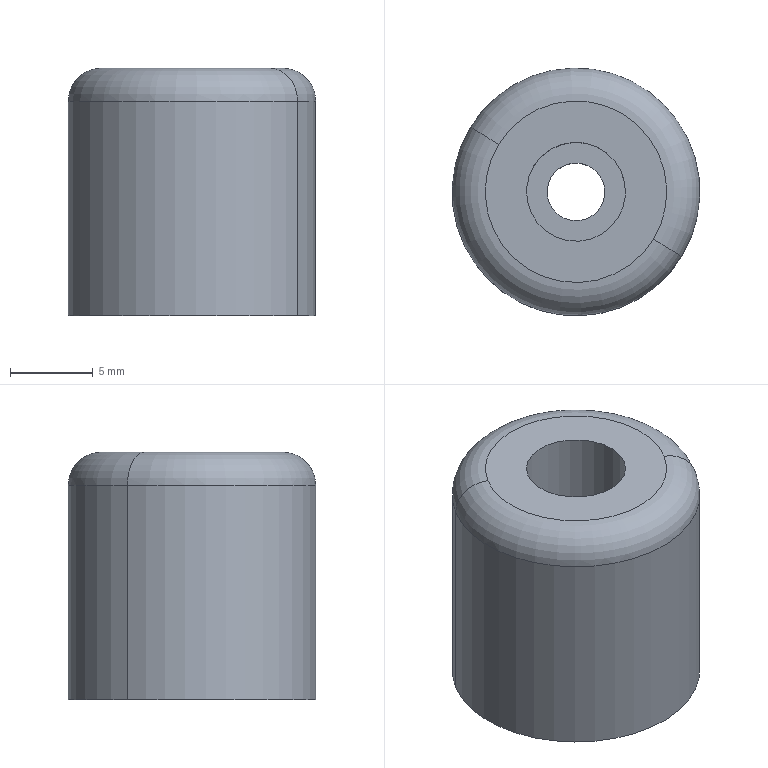Component | SolidWorks | DZ.KX.203-TC1505-20-18-05-92-1 | 1 solid | 14 faces | box 15 x 15 x 15 mm | volume 2153 mm3 | cylinder 8 | plane 4 | torus 2 | commonest cylinder face diameters 6 x2 3.5 x2 8 x2 15 x2 | material Plain Carbon Steel
build123d program:
from build123d import *

# Parameters (mm, degrees)
SKETCH1_R                                         = 7.5
BOSS_EXTRUDE1_DEPTH                               = 15
F_8_0_8_DIAMETER_HOLE1_D                          = 8
F_8_0_8_DIAMETER_HOLE1_DEPTH                      = 5
HOLE_SIZE_ACCORDING_TO_HEXAGON_SOCKET_D           = 3.5
HOLE_SIZE_ACCORDING_TO_HEXAGON_SOCKET_CBORE_D     = 6
HOLE_SIZE_ACCORDING_TO_HEXAGON_SOCKET_CBORE_DEPTH = 6
FILLET1_R                                         = 2


with BuildPart() as part:
    # Sketch1 → Boss-Extrude1 (new body)
    with BuildSketch(Plane(origin=(0, 0, 0), x_dir=(0, 0, -1), z_dir=(1, 0, 0))):
        Circle(SKETCH1_R)
    extrude(amount=BOSS_EXTRUDE1_DEPTH)

    # 8.0 _8_ Diameter Hole1
    with Locations(Plane(origin=(15, 0, 0), x_dir=(0, 0, -1), z_dir=(1, 0, 0))):
        with Locations((0, 0)):
            Hole(F_8_0_8_DIAMETER_HOLE1_D / 2, depth=F_8_0_8_DIAMETER_HOLE1_DEPTH)

    # Hole Size _according to_ Hexagon Socket (through all)
    with Locations(Plane.ZY):
        with Locations((0, 0)):
            CounterBoreHole(HOLE_SIZE_ACCORDING_TO_HEXAGON_SOCKET_D / 2, HOLE_SIZE_ACCORDING_TO_HEXAGON_SOCKET_CBORE_D / 2, HOLE_SIZE_ACCORDING_TO_HEXAGON_SOCKET_CBORE_DEPTH)

    # Fillet1
    fillet1_edges = [part.edges().sort_by_distance(p)[0] for p in [
        (0, 0, 7.5),
    ]]
    fillet(fillet1_edges, radius=FILLET1_R)


solid = part.part

# Placed as in the assembly
solid = solid.moved(Location((295.5, -817.807, 148.06), (0, 90, 0)))
STEP:
#1=COLOUR_RGB('',0.7922,0.8196,0.9333);
#2=FILL_AREA_STYLE_COLOUR('',#1);
#3=FILL_AREA_STYLE('',(#2));
#4=SURFACE_STYLE_FILL_AREA(#3);
#5=SURFACE_SIDE_STYLE('',(#4));
#6=SURFACE_STYLE_USAGE(.BOTH.,#5);
#7=PRESENTATION_STYLE_ASSIGNMENT((#6));
#8=CARTESIAN_POINT('',(11.819,-32.31,5.829));
#9=VERTEX_POINT('',#8);
#10=CARTESIAN_POINT('',(11.449,-32.084,5.829));
#11=VERTEX_POINT('',#10);
#12=CARTESIAN_POINT('',(11.634,-32.197,5.829));
#13=DIRECTION('',(-0.,0.,1.));
#14=DIRECTION('',(-0.8531,0.5218,0.));
#15=AXIS2_PLACEMENT_3D('',#12,#13,#14);
#16=CIRCLE('',#15,0.2165);
#17=EDGE_CURVE('',#9,#11,#16,.T.);
#18=ORIENTED_EDGE('',*,*,#17,.F.);
#19=CARTESIAN_POINT('',(11.886,-32.351,5.75));
#20=VERTEX_POINT('',#19);
#21=CARTESIAN_POINT('',(11.819,-32.31,5.75));
#22=DIRECTION('',(0.5218,0.8531,-0.));
#23=DIRECTION('',(-0.8531,0.5218,0.));
#24=AXIS2_PLACEMENT_3D('',#21,#22,#23);
#25=CIRCLE('',#24,0.07874);
#26=EDGE_CURVE('',#9,#20,#25,.T.);
#27=ORIENTED_EDGE('',*,*,#26,.T.);
#28=CARTESIAN_POINT('',(11.382,-32.043,5.75));
#29=VERTEX_POINT('',#28);
#30=CARTESIAN_POINT('',(11.634,-32.197,5.75));
#31=DIRECTION('',(0.,-0.,-1.));
#32=DIRECTION('',(-0.8531,0.5218,0.));
#33=AXIS2_PLACEMENT_3D('',#30,#31,#32);
#34=CIRCLE('',#33,0.2953);
#35=EDGE_CURVE('',#29,#20,#34,.T.);
#36=ORIENTED_EDGE('',*,*,#35,.F.);
#37=CARTESIAN_POINT('',(11.449,-32.084,5.75));
#38=DIRECTION('',(-0.5218,-0.8531,0.));
#39=DIRECTION('',(0.8531,-0.5218,0.));
#40=AXIS2_PLACEMENT_3D('',#37,#38,#39);
#41=CIRCLE('',#40,0.07874);
#42=EDGE_CURVE('',#11,#29,#41,.T.);
#43=ORIENTED_EDGE('',*,*,#42,.F.);
#44=EDGE_LOOP('',(#18,#27,#36,#43));
#45=FACE_OUTER_BOUND('',#44,.T.);
#46=CARTESIAN_POINT('',(11.634,-32.197,5.75));
#47=DIRECTION('',(0.,-0.,-1.));
#48=DIRECTION('',(-0.8531,0.5218,-0.));
#49=AXIS2_PLACEMENT_3D('',#46,#47,#48);
#50=TOROIDAL_SURFACE('',#49,0.2165,0.07874);
#51=ADVANCED_FACE('',(#45),#50,.T.);
#52=CARTESIAN_POINT('',(11.533,-32.135,5.593));
#53=VERTEX_POINT('',#52);
#54=CARTESIAN_POINT('',(11.735,-32.259,5.593));
#55=VERTEX_POINT('',#54);
#56=CARTESIAN_POINT('',(11.634,-32.197,5.593));
#57=DIRECTION('',(-0.,0.,1.));
#58=DIRECTION('',(0.8531,-0.5218,0.));
#59=AXIS2_PLACEMENT_3D('',#56,#57,#58);
#60=CIRCLE('',#59,0.1181);
#61=EDGE_CURVE('',#53,#55,#60,.T.);
#62=ORIENTED_EDGE('',*,*,#61,.F.);
#63=CARTESIAN_POINT('',(11.533,-32.135,5.829));
#64=VERTEX_POINT('',#63);
#65=CARTESIAN_POINT('',(11.533,-32.135,5.829));
#66=DIRECTION('',(-0.,0.,1.));
#67=VECTOR('',#66,39.37);
#68=LINE('',#65,#67);
#69=EDGE_CURVE('',#53,#64,#68,.T.);
#70=ORIENTED_EDGE('',*,*,#69,.T.);
#71=CARTESIAN_POINT('',(11.735,-32.259,5.829));
#72=VERTEX_POINT('',#71);
#73=CARTESIAN_POINT('',(11.634,-32.197,5.829));
#74=DIRECTION('',(-0.,0.,1.));
#75=DIRECTION('',(0.8531,-0.5218,0.));
#76=AXIS2_PLACEMENT_3D('',#73,#74,#75);
#77=CIRCLE('',#76,0.1181);
#78=EDGE_CURVE('',#64,#72,#77,.T.);
#79=ORIENTED_EDGE('',*,*,#78,.T.);
#80=CARTESIAN_POINT('',(11.735,-32.259,5.829));
#81=DIRECTION('',(-0.,0.,1.));
#82=VECTOR('',#81,39.37);
#83=LINE('',#80,#82);
#84=EDGE_CURVE('',#55,#72,#83,.T.);
#85=ORIENTED_EDGE('',*,*,#84,.F.);
#86=EDGE_LOOP('',(#62,#70,#79,#85));
#87=FACE_OUTER_BOUND('',#86,.T.);
#88=CARTESIAN_POINT('',(11.634,-32.197,5.829));
#89=DIRECTION('',(-0.,0.,1.));
#90=DIRECTION('',(0.8531,-0.5218,0.));
#91=AXIS2_PLACEMENT_3D('',#88,#89,#90);
#92=CYLINDRICAL_SURFACE('',#91,0.1181);
#93=ADVANCED_FACE('',(#87),#92,.F.);
#94=CARTESIAN_POINT('',(11.575,-32.161,5.435));
#95=VERTEX_POINT('',#94);
#96=CARTESIAN_POINT('',(11.693,-32.233,5.435));
#97=VERTEX_POINT('',#96);
#98=CARTESIAN_POINT('',(11.634,-32.197,5.435));
#99=DIRECTION('',(-0.,0.,1.));
#100=DIRECTION('',(0.8531,-0.5218,0.));
#101=AXIS2_PLACEMENT_3D('',#98,#99,#100);
#102=CIRCLE('',#101,0.0689);
#103=EDGE_CURVE('',#95,#97,#102,.T.);
#104=ORIENTED_EDGE('',*,*,#103,.F.);
#105=CARTESIAN_POINT('',(11.575,-32.161,5.593));
#106=VERTEX_POINT('',#105);
#107=CARTESIAN_POINT('',(11.575,-32.161,5.829));
#108=DIRECTION('',(-0.,0.,1.));
#109=VECTOR('',#108,39.37);
#110=LINE('',#107,#109);
#111=EDGE_CURVE('',#95,#106,#110,.T.);
#112=ORIENTED_EDGE('',*,*,#111,.T.);
#113=CARTESIAN_POINT('',(11.693,-32.233,5.593));
#114=VERTEX_POINT('',#113);
#115=CARTESIAN_POINT('',(11.634,-32.197,5.593));
#116=DIRECTION('',(-0.,0.,1.));
#117=DIRECTION('',(0.8531,-0.5218,0.));
#118=AXIS2_PLACEMENT_3D('',#115,#116,#117);
#119=CIRCLE('',#118,0.0689);
#120=EDGE_CURVE('',#106,#114,#119,.T.);
#121=ORIENTED_EDGE('',*,*,#120,.T.);
#122=CARTESIAN_POINT('',(11.693,-32.233,5.829));
#123=DIRECTION('',(-0.,0.,1.));
#124=VECTOR('',#123,39.37);
#125=LINE('',#122,#124);
#126=EDGE_CURVE('',#97,#114,#125,.T.);
#127=ORIENTED_EDGE('',*,*,#126,.F.);
#128=EDGE_LOOP('',(#104,#112,#121,#127));
#129=FACE_OUTER_BOUND('',#128,.T.);
#130=CARTESIAN_POINT('',(11.634,-32.197,5.829));
#131=DIRECTION('',(-0.,0.,1.));
#132=DIRECTION('',(0.8531,-0.5218,0.));
#133=AXIS2_PLACEMENT_3D('',#130,#131,#132);
#134=CYLINDRICAL_SURFACE('',#133,0.0689);
#135=ADVANCED_FACE('',(#129),#134,.F.);
#136=CARTESIAN_POINT('',(11.768,-32.279,5.435));
#137=VERTEX_POINT('',#136);
#138=CARTESIAN_POINT('',(11.5,-32.115,5.435));
#139=VERTEX_POINT('',#138);
#140=CARTESIAN_POINT('',(11.634,-32.197,5.435));
#141=DIRECTION('',(0.,-0.,-1.));
#142=DIRECTION('',(-0.8531,0.5218,0.));
#143=AXIS2_PLACEMENT_3D('',#140,#141,#142);
#144=CIRCLE('',#143,0.1575);
#145=EDGE_CURVE('',#137,#139,#144,.T.);
#146=ORIENTED_EDGE('',*,*,#145,.F.);
#147=CARTESIAN_POINT('',(11.768,-32.279,5.239));
#148=VERTEX_POINT('',#147);
#149=CARTESIAN_POINT('',(11.768,-32.279,5.239));
#150=DIRECTION('',(0.,-0.,-1.));
#151=VECTOR('',#150,39.37);
#152=LINE('',#149,#151);
#153=EDGE_CURVE('',#137,#148,#152,.T.);
#154=ORIENTED_EDGE('',*,*,#153,.T.);
#155=CARTESIAN_POINT('',(11.5,-32.115,5.239));
#156=VERTEX_POINT('',#155);
#157=CARTESIAN_POINT('',(11.634,-32.197,5.239));
#158=DIRECTION('',(0.,-0.,-1.));
#159=DIRECTION('',(-0.8531,0.5218,0.));
#160=AXIS2_PLACEMENT_3D('',#157,#158,#159);
#161=CIRCLE('',#160,0.1575);
#162=EDGE_CURVE('',#148,#156,#161,.T.);
#163=ORIENTED_EDGE('',*,*,#162,.T.);
#164=CARTESIAN_POINT('',(11.5,-32.115,5.239));
#165=DIRECTION('',(0.,-0.,-1.));
#166=VECTOR('',#165,39.37);
#167=LINE('',#164,#166);
#168=EDGE_CURVE('',#139,#156,#167,.T.);
#169=ORIENTED_EDGE('',*,*,#168,.F.);
#170=EDGE_LOOP('',(#146,#154,#163,#169));
#171=FACE_OUTER_BOUND('',#170,.T.);
#172=CARTESIAN_POINT('',(11.634,-32.197,5.239));
#173=DIRECTION('',(0.,-0.,-1.));
#174=DIRECTION('',(-0.8531,0.5218,0.));
#175=AXIS2_PLACEMENT_3D('',#172,#173,#174);
#176=CYLINDRICAL_SURFACE('',#175,0.1575);
#177=ADVANCED_FACE('',(#171),#176,.F.);
#178=CARTESIAN_POINT('',(11.382,-32.043,5.239));
#179=VERTEX_POINT('',#178);
#180=CARTESIAN_POINT('',(11.886,-32.351,5.239));
#181=VERTEX_POINT('',#180);
#182=CARTESIAN_POINT('',(11.634,-32.197,5.239));
#183=DIRECTION('',(0.,-0.,-1.));
#184=DIRECTION('',(-0.8531,0.5218,0.));
#185=AXIS2_PLACEMENT_3D('',#182,#183,#184);
#186=CIRCLE('',#185,0.2953);
#187=EDGE_CURVE('',#179,#181,#186,.T.);
#188=ORIENTED_EDGE('',*,*,#187,.F.);
#189=CARTESIAN_POINT('',(11.382,-32.043,5.239));
#190=DIRECTION('',(-0.,0.,1.));
#191=VECTOR('',#190,39.37);
#192=LINE('',#189,#191);
#193=EDGE_CURVE('',#179,#29,#192,.T.);
#194=ORIENTED_EDGE('',*,*,#193,.T.);
#195=ORIENTED_EDGE('',*,*,#35,.T.);
#196=CARTESIAN_POINT('',(11.886,-32.351,5.239));
#197=DIRECTION('',(-0.,0.,1.));
#198=VECTOR('',#197,39.37);
#199=LINE('',#196,#198);
#200=EDGE_CURVE('',#181,#20,#199,.T.);
#201=ORIENTED_EDGE('',*,*,#200,.F.);
#202=EDGE_LOOP('',(#188,#194,#195,#201));
#203=FACE_OUTER_BOUND('',#202,.T.);
#204=CARTESIAN_POINT('',(11.634,-32.197,5.239));
#205=DIRECTION('',(-0.,0.,1.));
#206=DIRECTION('',(0.8531,-0.5218,0.));
#207=AXIS2_PLACEMENT_3D('',#204,#205,#206);
#208=CYLINDRICAL_SURFACE('',#207,0.2953);
#209=ADVANCED_FACE('',(#203),#208,.T.);
#210=ORIENTED_EDGE('',*,*,#193,.F.);
#211=CARTESIAN_POINT('',(11.634,-32.197,5.239));
#212=DIRECTION('',(0.,-0.,-1.));
#213=DIRECTION('',(-0.8531,0.5218,0.));
#214=AXIS2_PLACEMENT_3D('',#211,#212,#213);
#215=CIRCLE('',#214,0.2953);
#216=EDGE_CURVE('',#181,#179,#215,.T.);
#217=ORIENTED_EDGE('',*,*,#216,.F.);
#218=ORIENTED_EDGE('',*,*,#200,.T.);
#219=CARTESIAN_POINT('',(11.634,-32.197,5.75));
#220=DIRECTION('',(0.,-0.,-1.));
#221=DIRECTION('',(-0.8531,0.5218,0.));
#222=AXIS2_PLACEMENT_3D('',#219,#220,#221);
#223=CIRCLE('',#222,0.2953);
#224=EDGE_CURVE('',#20,#29,#223,.T.);
#225=ORIENTED_EDGE('',*,*,#224,.T.);
#226=EDGE_LOOP('',(#210,#217,#218,#225));
#227=FACE_OUTER_BOUND('',#226,.T.);
#228=CARTESIAN_POINT('',(11.634,-32.197,5.239));
#229=DIRECTION('',(-0.,0.,1.));
#230=DIRECTION('',(0.8531,-0.5218,0.));
#231=AXIS2_PLACEMENT_3D('',#228,#229,#230);
#232=CYLINDRICAL_SURFACE('',#231,0.2953);
#233=ADVANCED_FACE('',(#227),#232,.T.);
#234=CARTESIAN_POINT('',(11.634,-32.197,5.239));
#235=DIRECTION('',(0.,-0.,-1.));
#236=DIRECTION('',(-0.8531,0.5218,0.));
#237=AXIS2_PLACEMENT_3D('',#234,#235,#236);
#238=CIRCLE('',#237,0.1575);
#239=EDGE_CURVE('',#156,#148,#238,.T.);
#240=ORIENTED_EDGE('',*,*,#239,.F.);
#241=ORIENTED_EDGE('',*,*,#162,.F.);
#242=EDGE_LOOP('',(#240,#241));
#243=FACE_BOUND('',#242,.T.);
#244=ORIENTED_EDGE('',*,*,#216,.T.);
#245=ORIENTED_EDGE('',*,*,#187,.T.);
#246=EDGE_LOOP('',(#244,#245));
#247=FACE_OUTER_BOUND('',#246,.T.);
#248=CARTESIAN_POINT('',(11.634,-32.197,5.239));
#249=DIRECTION('',(0.,-0.,-1.));
#250=DIRECTION('',(-0.8531,0.5218,-0.));
#251=AXIS2_PLACEMENT_3D('',#248,#249,#250);
#252=PLANE('',#251);
#253=ADVANCED_FACE('',(#243,#247),#252,.T.);
#254=CARTESIAN_POINT('',(11.634,-32.197,5.829));
#255=DIRECTION('',(-0.,0.,1.));
#256=DIRECTION('',(-0.8531,0.5218,0.));
#257=AXIS2_PLACEMENT_3D('',#254,#255,#256);
#258=CIRCLE('',#257,0.2165);
#259=EDGE_CURVE('',#11,#9,#258,.T.);
#260=ORIENTED_EDGE('',*,*,#259,.T.);
#261=ORIENTED_EDGE('',*,*,#17,.T.);
#262=EDGE_LOOP('',(#260,#261));
#263=FACE_OUTER_BOUND('',#262,.T.);
#264=CARTESIAN_POINT('',(11.634,-32.197,5.829));
#265=DIRECTION('',(-0.,0.,1.));
#266=DIRECTION('',(0.8531,-0.5218,0.));
#267=AXIS2_PLACEMENT_3D('',#264,#265,#266);
#268=CIRCLE('',#267,0.1181);
#269=EDGE_CURVE('',#72,#64,#268,.T.);
#270=ORIENTED_EDGE('',*,*,#269,.F.);
#271=ORIENTED_EDGE('',*,*,#78,.F.);
#272=EDGE_LOOP('',(#270,#271));
#273=FACE_BOUND('',#272,.T.);
#274=CARTESIAN_POINT('',(11.634,-32.197,5.829));
#275=DIRECTION('',(0.,-0.,-1.));
#276=DIRECTION('',(-0.8531,0.5218,-0.));
#277=AXIS2_PLACEMENT_3D('',#274,#275,#276);
#278=PLANE('',#277);
#279=ADVANCED_FACE('',(#263,#273),#278,.F.);
#280=CARTESIAN_POINT('',(11.634,-32.197,5.435));
#281=DIRECTION('',(-0.,0.,1.));
#282=DIRECTION('',(0.8531,-0.5218,0.));
#283=AXIS2_PLACEMENT_3D('',#280,#281,#282);
#284=CIRCLE('',#283,0.0689);
#285=EDGE_CURVE('',#97,#95,#284,.T.);
#286=ORIENTED_EDGE('',*,*,#285,.T.);
#287=ORIENTED_EDGE('',*,*,#103,.T.);
#288=EDGE_LOOP('',(#286,#287));
#289=FACE_BOUND('',#288,.T.);
#290=CARTESIAN_POINT('',(11.634,-32.197,5.435));
#291=DIRECTION('',(0.,-0.,-1.));
#292=DIRECTION('',(-0.8531,0.5218,0.));
#293=AXIS2_PLACEMENT_3D('',#290,#291,#292);
#294=CIRCLE('',#293,0.1575);
#295=EDGE_CURVE('',#139,#137,#294,.T.);
#296=ORIENTED_EDGE('',*,*,#295,.T.);
#297=ORIENTED_EDGE('',*,*,#145,.T.);
#298=EDGE_LOOP('',(#296,#297));
#299=FACE_OUTER_BOUND('',#298,.T.);
#300=CARTESIAN_POINT('',(11.634,-32.197,5.435));
#301=DIRECTION('',(-0.,0.,1.));
#302=DIRECTION('',(0.8531,-0.5218,0.));
#303=AXIS2_PLACEMENT_3D('',#300,#301,#302);
#304=PLANE('',#303);
#305=ADVANCED_FACE('',(#289,#299),#304,.F.);
#306=ORIENTED_EDGE('',*,*,#153,.F.);
#307=ORIENTED_EDGE('',*,*,#295,.F.);
#308=ORIENTED_EDGE('',*,*,#168,.T.);
#309=ORIENTED_EDGE('',*,*,#239,.T.);
#310=EDGE_LOOP('',(#306,#307,#308,#309));
#311=FACE_OUTER_BOUND('',#310,.T.);
#312=CARTESIAN_POINT('',(11.634,-32.197,5.239));
#313=DIRECTION('',(0.,-0.,-1.));
#314=DIRECTION('',(-0.8531,0.5218,0.));
#315=AXIS2_PLACEMENT_3D('',#312,#313,#314);
#316=CYLINDRICAL_SURFACE('',#315,0.1575);
#317=ADVANCED_FACE('',(#311),#316,.F.);
#318=ORIENTED_EDGE('',*,*,#111,.F.);
#319=ORIENTED_EDGE('',*,*,#285,.F.);
#320=ORIENTED_EDGE('',*,*,#126,.T.);
#321=CARTESIAN_POINT('',(11.634,-32.197,5.593));
#322=DIRECTION('',(-0.,0.,1.));
#323=DIRECTION('',(0.8531,-0.5218,0.));
#324=AXIS2_PLACEMENT_3D('',#321,#322,#323);
#325=CIRCLE('',#324,0.0689);
#326=EDGE_CURVE('',#114,#106,#325,.T.);
#327=ORIENTED_EDGE('',*,*,#326,.T.);
#328=EDGE_LOOP('',(#318,#319,#320,#327));
#329=FACE_OUTER_BOUND('',#328,.T.);
#330=CARTESIAN_POINT('',(11.634,-32.197,5.829));
#331=DIRECTION('',(-0.,0.,1.));
#332=DIRECTION('',(0.8531,-0.5218,0.));
#333=AXIS2_PLACEMENT_3D('',#330,#331,#332);
#334=CYLINDRICAL_SURFACE('',#333,0.0689);
#335=ADVANCED_FACE('',(#329),#334,.F.);
#336=ORIENTED_EDGE('',*,*,#326,.F.);
#337=ORIENTED_EDGE('',*,*,#120,.F.);
#338=EDGE_LOOP('',(#336,#337));
#339=FACE_BOUND('',#338,.T.);
#340=CARTESIAN_POINT('',(11.634,-32.197,5.593));
#341=DIRECTION('',(-0.,0.,1.));
#342=DIRECTION('',(0.8531,-0.5218,0.));
#343=AXIS2_PLACEMENT_3D('',#340,#341,#342);
#344=CIRCLE('',#343,0.1181);
#345=EDGE_CURVE('',#55,#53,#344,.T.);
#346=ORIENTED_EDGE('',*,*,#345,.T.);
#347=ORIENTED_EDGE('',*,*,#61,.T.);
#348=EDGE_LOOP('',(#346,#347));
#349=FACE_OUTER_BOUND('',#348,.T.);
#350=CARTESIAN_POINT('',(11.67,-32.138,5.593));
#351=DIRECTION('',(0.,-0.,-1.));
#352=DIRECTION('',(-0.8531,0.5218,-0.));
#353=AXIS2_PLACEMENT_3D('',#350,#351,#352);
#354=PLANE('',#353);
#355=ADVANCED_FACE('',(#339,#349),#354,.F.);
#356=ORIENTED_EDGE('',*,*,#69,.F.);
#357=ORIENTED_EDGE('',*,*,#345,.F.);
#358=ORIENTED_EDGE('',*,*,#84,.T.);
#359=ORIENTED_EDGE('',*,*,#269,.T.);
#360=EDGE_LOOP('',(#356,#357,#358,#359));
#361=FACE_OUTER_BOUND('',#360,.T.);
#362=CARTESIAN_POINT('',(11.634,-32.197,5.829));
#363=DIRECTION('',(-0.,0.,1.));
#364=DIRECTION('',(0.8531,-0.5218,0.));
#365=AXIS2_PLACEMENT_3D('',#362,#363,#364);
#366=CYLINDRICAL_SURFACE('',#365,0.1181);
#367=ADVANCED_FACE('',(#361),#366,.F.);
#368=ORIENTED_EDGE('',*,*,#26,.F.);
#369=ORIENTED_EDGE('',*,*,#259,.F.);
#370=ORIENTED_EDGE('',*,*,#42,.T.);
#371=ORIENTED_EDGE('',*,*,#224,.F.);
#372=EDGE_LOOP('',(#368,#369,#370,#371));
#373=FACE_OUTER_BOUND('',#372,.T.);
#374=CARTESIAN_POINT('',(11.634,-32.197,5.75));
#375=DIRECTION('',(0.,-0.,-1.));
#376=DIRECTION('',(-0.8531,0.5218,-0.));
#377=AXIS2_PLACEMENT_3D('',#374,#375,#376);
#378=TOROIDAL_SURFACE('',#377,0.2165,0.07874);
#379=ADVANCED_FACE('',(#373),#378,.T.);
#380=CLOSED_SHELL('',(#51,#93,#135,#177,#209,#233,#253,#279,#305,#317,#335,#355,#367,#379));
#381=MANIFOLD_SOLID_BREP('',#380);
#382=STYLED_ITEM('',(#7),#381);
#383=(LENGTH_UNIT()NAMED_UNIT(*)SI_UNIT($,.METRE.));
#384=LENGTH_MEASURE_WITH_UNIT(LENGTH_MEASURE(0.0254),#383);
#385=DIMENSIONAL_EXPONENTS(1.,0.,0.,0.,0.,0.,0.);
#386=(CONVERSION_BASED_UNIT('',#384)LENGTH_UNIT()NAMED_UNIT(#385));
#387=UNCERTAINTY_MEASURE_WITH_UNIT(LENGTH_MEASURE(0.00001),#386,'','');
#388=(NAMED_UNIT(*)PLANE_ANGLE_UNIT()SI_UNIT($,.RADIAN.));
#389=(NAMED_UNIT(*)SI_UNIT($,.STERADIAN.)SOLID_ANGLE_UNIT());
#390=(GEOMETRIC_REPRESENTATION_CONTEXT(3)GLOBAL_UNCERTAINTY_ASSIGNED_CONTEXT((#387))GLOBAL_UNIT_ASSIGNED_CONTEXT((#386,#388,#389))REPRESENTATION_CONTEXT('',''));
#391=MECHANICAL_DESIGN_GEOMETRIC_PRESENTATION_REPRESENTATION('',(#382),#390);
#392=CARTESIAN_POINT('',(0.,0.,0.));
#393=DIRECTION('',(0.,0.,1.));
#394=DIRECTION('',(1.,0.,0.));
#395=AXIS2_PLACEMENT_3D('',#392,#393,#394);
#396=(LENGTH_UNIT()NAMED_UNIT(*)SI_UNIT($,.METRE.));
#397=LENGTH_MEASURE_WITH_UNIT(LENGTH_MEASURE(0.0254),#396);
#398=DIMENSIONAL_EXPONENTS(1.,0.,0.,0.,0.,0.,0.);
#399=(CONVERSION_BASED_UNIT('',#397)LENGTH_UNIT()NAMED_UNIT(#398));
#400=UNCERTAINTY_MEASURE_WITH_UNIT(LENGTH_MEASURE(0.00001),#399,'','');
#401=(NAMED_UNIT(*)PLANE_ANGLE_UNIT()SI_UNIT($,.RADIAN.));
#402=(NAMED_UNIT(*)SI_UNIT($,.STERADIAN.)SOLID_ANGLE_UNIT());
#403=(GEOMETRIC_REPRESENTATION_CONTEXT(3)GLOBAL_UNCERTAINTY_ASSIGNED_CONTEXT((#400))GLOBAL_UNIT_ASSIGNED_CONTEXT((#399,#401,#402))REPRESENTATION_CONTEXT('',''));
#404=ADVANCED_BREP_SHAPE_REPRESENTATION('',(#381,#395),#403);
#405=PRESENTATION_LAYER_ASSIGNMENT('','',(#382));